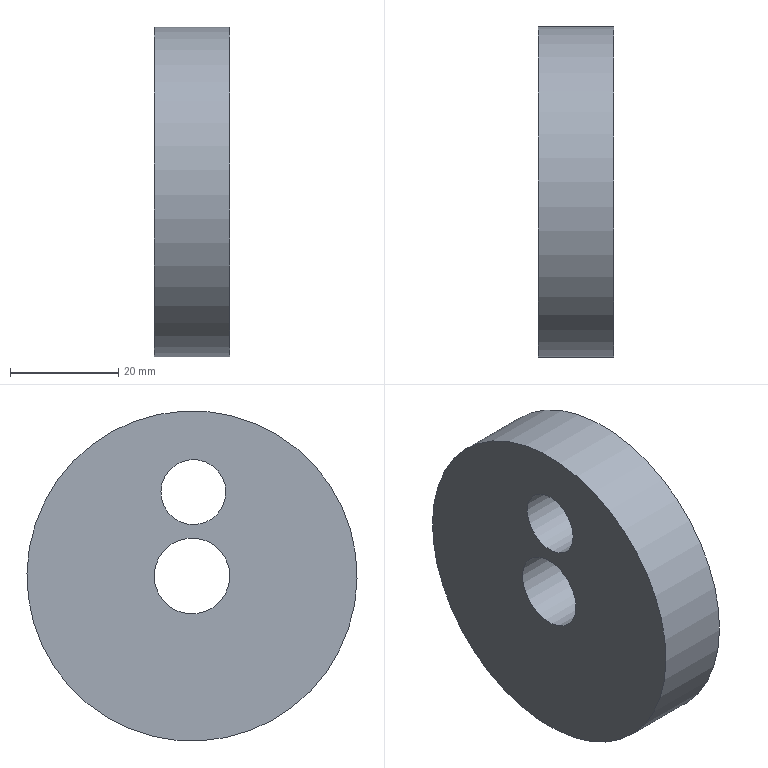Component | NX | CONNECTING_PLATE | 1 solid | 5 faces | box 14 x 61 x 61 mm | volume 37176 mm3 | cylinder 3 | plane 2 | commonest cylinder face diameters 12 x1 61 x1 14 x1
STEP:
#1=CARTESIAN_POINT('',(0.,0.,0.));
#2=DIRECTION('',(0.,0.,1.));
#3=DIRECTION('',(1.,0.,0.));
#4=AXIS2_PLACEMENT_3D('',#1,#2,#3);
#5=CARTESIAN_POINT('',(-95.,-6.249,138.401));
#6=VERTEX_POINT('',#5);
#7=CARTESIAN_POINT('',(-95.,-0.25,138.498));
#8=DIRECTION('',(-1.,0.,0.));
#9=DIRECTION('',(0.,-0.9999,-0.01613));
#10=AXIS2_PLACEMENT_3D('',#7,#8,#9);
#11=CIRCLE('',#10,6.);
#12=CARTESIAN_POINT('',(-95.,-0.25,138.498));
#13=DIRECTION('',(1.,0.,0.));
#14=DIRECTION('',(0.,0.9999,0.01613));
#15=AXIS2_PLACEMENT_3D('',#12,#13,#14);
#16=CYLINDRICAL_SURFACE('',#15,6.);
#17=CARTESIAN_POINT('',(9.425,0.));
#18=DIRECTION('',(-1.,0.));
#19=VECTOR('',#18,1.);
#20=LINE('',#17,#19);
#21=(GEOMETRIC_REPRESENTATION_CONTEXT(2)PARAMETRIC_REPRESENTATION_CONTEXT()REPRESENTATION_CONTEXT('',''));
#22=DEFINITIONAL_REPRESENTATION('',(#20),#21);
#23=PCURVE('',#16,#22);
#24=CARTESIAN_POINT('',(-95.,-0.125,130.749));
#25=DIRECTION('',(-1.,0.,0.));
#26=DIRECTION('',(0.,-0.9999,-0.01613));
#27=AXIS2_PLACEMENT_3D('',#24,#25,#26);
#28=PLANE('',#27);
#29=CARTESIAN_POINT('',(0.,7.75));
#30=DIRECTION('',(1.,-0.));
#31=AXIS2_PLACEMENT_2D('',#29,#30);
#32=CIRCLE('',#31,6.);
#33=(GEOMETRIC_REPRESENTATION_CONTEXT(2)PARAMETRIC_REPRESENTATION_CONTEXT()REPRESENTATION_CONTEXT('',''));
#34=DEFINITIONAL_REPRESENTATION('',(#32),#33);
#35=PCURVE('',#28,#34);
#36=SURFACE_CURVE('',#11,(#23,#35),.PCURVE_S1.);
#37=EDGE_CURVE('',#6,#6,#36,.T.);
#38=ORIENTED_EDGE('',*,*,#37,.F.);
#39=CARTESIAN_POINT('',(-81.,-6.249,138.401));
#40=VERTEX_POINT('',#39);
#41=CARTESIAN_POINT('',(-95.,-6.249,138.401));
#42=CARTESIAN_POINT('',(-81.,-6.249,138.401));
#43=B_SPLINE_CURVE_WITH_KNOTS('',1,(#41,#42),.UNSPECIFIED.,.F.,.F.,(2,2),(0.,14.),.PIECEWISE_BEZIER_KNOTS.);
#44=CARTESIAN_POINT('',(9.425,0.));
#45=DIRECTION('',(0.,1.));
#46=VECTOR('',#45,1.);
#47=LINE('',#44,#46);
#48=(GEOMETRIC_REPRESENTATION_CONTEXT(2)PARAMETRIC_REPRESENTATION_CONTEXT()REPRESENTATION_CONTEXT('',''));
#49=DEFINITIONAL_REPRESENTATION('',(#47),#48);
#50=PCURVE('',#16,#49);
#51=CARTESIAN_POINT('',(3.142,0.));
#52=DIRECTION('',(0.,1.));
#53=VECTOR('',#52,1.);
#54=LINE('',#51,#53);
#55=(GEOMETRIC_REPRESENTATION_CONTEXT(2)PARAMETRIC_REPRESENTATION_CONTEXT()REPRESENTATION_CONTEXT('',''));
#56=DEFINITIONAL_REPRESENTATION('',(#54),#55);
#57=PCURVE('',#16,#56);
#58=SEAM_CURVE('',#43,(#50,#57),.PCURVE_S1.);
#59=EDGE_CURVE('',#6,#40,#58,.T.);
#60=ORIENTED_EDGE('',*,*,#59,.T.);
#61=CARTESIAN_POINT('',(-81.,-0.25,138.498));
#62=DIRECTION('',(-1.,0.,0.));
#63=DIRECTION('',(0.,-0.9999,-0.01613));
#64=AXIS2_PLACEMENT_3D('',#61,#62,#63);
#65=CIRCLE('',#64,6.);
#66=CARTESIAN_POINT('',(9.425,14.));
#67=DIRECTION('',(-1.,0.));
#68=VECTOR('',#67,1.);
#69=LINE('',#66,#68);
#70=(GEOMETRIC_REPRESENTATION_CONTEXT(2)PARAMETRIC_REPRESENTATION_CONTEXT()REPRESENTATION_CONTEXT('',''));
#71=DEFINITIONAL_REPRESENTATION('',(#69),#70);
#72=PCURVE('',#16,#71);
#73=CARTESIAN_POINT('',(-81.,-0.125,130.749));
#74=DIRECTION('',(-1.,0.,0.));
#75=DIRECTION('',(0.,-0.9999,-0.01613));
#76=AXIS2_PLACEMENT_3D('',#73,#74,#75);
#77=PLANE('',#76);
#78=CARTESIAN_POINT('',(0.,7.75));
#79=DIRECTION('',(1.,-0.));
#80=AXIS2_PLACEMENT_2D('',#78,#79);
#81=CIRCLE('',#80,6.);
#82=(GEOMETRIC_REPRESENTATION_CONTEXT(2)PARAMETRIC_REPRESENTATION_CONTEXT()REPRESENTATION_CONTEXT('',''));
#83=DEFINITIONAL_REPRESENTATION('',(#81),#82);
#84=PCURVE('',#77,#83);
#85=SURFACE_CURVE('',#65,(#72,#84),.PCURVE_S1.);
#86=EDGE_CURVE('',#40,#40,#85,.T.);
#87=ORIENTED_EDGE('',*,*,#86,.T.);
#88=ORIENTED_EDGE('',*,*,#59,.F.);
#89=EDGE_LOOP('',(#38,#60,#87,#88));
#90=FACE_BOUND('',#89,.F.);
#91=ADVANCED_FACE('',(#90),#16,.F.);
#92=CARTESIAN_POINT('',(-95.,-30.496,122.508));
#93=VERTEX_POINT('',#92);
#94=CARTESIAN_POINT('',(-95.,-0.,123.));
#95=DIRECTION('',(-1.,0.,0.));
#96=DIRECTION('',(0.,-0.9999,-0.01613));
#97=AXIS2_PLACEMENT_3D('',#94,#95,#96);
#98=CIRCLE('',#97,30.5);
#99=CARTESIAN_POINT('',(-95.,-0.,123.));
#100=DIRECTION('',(1.,0.,0.));
#101=DIRECTION('',(0.,0.9999,0.01613));
#102=AXIS2_PLACEMENT_3D('',#99,#100,#101);
#103=CYLINDRICAL_SURFACE('',#102,30.5);
#104=CARTESIAN_POINT('',(9.425,0.));
#105=DIRECTION('',(-1.,0.));
#106=VECTOR('',#105,1.);
#107=LINE('',#104,#106);
#108=(GEOMETRIC_REPRESENTATION_CONTEXT(2)PARAMETRIC_REPRESENTATION_CONTEXT()REPRESENTATION_CONTEXT('',''));
#109=DEFINITIONAL_REPRESENTATION('',(#107),#108);
#110=PCURVE('',#103,#109);
#111=CARTESIAN_POINT('',(0.,-7.75));
#112=DIRECTION('',(1.,0.));
#113=AXIS2_PLACEMENT_2D('',#111,#112);
#114=CIRCLE('',#113,30.5);
#115=(GEOMETRIC_REPRESENTATION_CONTEXT(2)PARAMETRIC_REPRESENTATION_CONTEXT()REPRESENTATION_CONTEXT('',''));
#116=DEFINITIONAL_REPRESENTATION('',(#114),#115);
#117=PCURVE('',#28,#116);
#118=SURFACE_CURVE('',#98,(#110,#117),.PCURVE_S1.);
#119=EDGE_CURVE('',#93,#93,#118,.T.);
#120=ORIENTED_EDGE('',*,*,#119,.F.);
#121=CARTESIAN_POINT('',(-81.,-30.496,122.508));
#122=VERTEX_POINT('',#121);
#123=CARTESIAN_POINT('',(-95.,-30.496,122.508));
#124=CARTESIAN_POINT('',(-81.,-30.496,122.508));
#125=B_SPLINE_CURVE_WITH_KNOTS('',1,(#123,#124),.UNSPECIFIED.,.F.,.F.,(2,2),(0.,14.),.PIECEWISE_BEZIER_KNOTS.);
#126=CARTESIAN_POINT('',(9.425,0.));
#127=DIRECTION('',(0.,1.));
#128=VECTOR('',#127,1.);
#129=LINE('',#126,#128);
#130=(GEOMETRIC_REPRESENTATION_CONTEXT(2)PARAMETRIC_REPRESENTATION_CONTEXT()REPRESENTATION_CONTEXT('',''));
#131=DEFINITIONAL_REPRESENTATION('',(#129),#130);
#132=PCURVE('',#103,#131);
#133=CARTESIAN_POINT('',(3.142,0.));
#134=DIRECTION('',(0.,1.));
#135=VECTOR('',#134,1.);
#136=LINE('',#133,#135);
#137=(GEOMETRIC_REPRESENTATION_CONTEXT(2)PARAMETRIC_REPRESENTATION_CONTEXT()REPRESENTATION_CONTEXT('',''));
#138=DEFINITIONAL_REPRESENTATION('',(#136),#137);
#139=PCURVE('',#103,#138);
#140=SEAM_CURVE('',#125,(#132,#139),.PCURVE_S1.);
#141=EDGE_CURVE('',#93,#122,#140,.T.);
#142=ORIENTED_EDGE('',*,*,#141,.T.);
#143=CARTESIAN_POINT('',(-81.,-0.,123.));
#144=DIRECTION('',(-1.,0.,0.));
#145=DIRECTION('',(0.,-0.9999,-0.01613));
#146=AXIS2_PLACEMENT_3D('',#143,#144,#145);
#147=CIRCLE('',#146,30.5);
#148=CARTESIAN_POINT('',(9.425,14.));
#149=DIRECTION('',(-1.,0.));
#150=VECTOR('',#149,1.);
#151=LINE('',#148,#150);
#152=(GEOMETRIC_REPRESENTATION_CONTEXT(2)PARAMETRIC_REPRESENTATION_CONTEXT()REPRESENTATION_CONTEXT('',''));
#153=DEFINITIONAL_REPRESENTATION('',(#151),#152);
#154=PCURVE('',#103,#153);
#155=CARTESIAN_POINT('',(0.,-7.75));
#156=DIRECTION('',(1.,0.));
#157=AXIS2_PLACEMENT_2D('',#155,#156);
#158=CIRCLE('',#157,30.5);
#159=(GEOMETRIC_REPRESENTATION_CONTEXT(2)PARAMETRIC_REPRESENTATION_CONTEXT()REPRESENTATION_CONTEXT('',''));
#160=DEFINITIONAL_REPRESENTATION('',(#158),#159);
#161=PCURVE('',#77,#160);
#162=SURFACE_CURVE('',#147,(#154,#161),.PCURVE_S1.);
#163=EDGE_CURVE('',#122,#122,#162,.T.);
#164=ORIENTED_EDGE('',*,*,#163,.T.);
#165=ORIENTED_EDGE('',*,*,#141,.F.);
#166=EDGE_LOOP('',(#120,#142,#164,#165));
#167=FACE_BOUND('',#166,.T.);
#168=ADVANCED_FACE('',(#167),#103,.T.);
#169=CARTESIAN_POINT('',(-95.,-6.999,122.887));
#170=VERTEX_POINT('',#169);
#171=CARTESIAN_POINT('',(-95.,-0.,123.));
#172=DIRECTION('',(-1.,0.,0.));
#173=DIRECTION('',(0.,-0.9999,-0.01613));
#174=AXIS2_PLACEMENT_3D('',#171,#172,#173);
#175=CIRCLE('',#174,7.);
#176=CARTESIAN_POINT('',(-95.,-0.,123.));
#177=DIRECTION('',(1.,0.,0.));
#178=DIRECTION('',(0.,0.9999,0.01613));
#179=AXIS2_PLACEMENT_3D('',#176,#177,#178);
#180=CYLINDRICAL_SURFACE('',#179,7.);
#181=CARTESIAN_POINT('',(9.425,0.));
#182=DIRECTION('',(-1.,0.));
#183=VECTOR('',#182,1.);
#184=LINE('',#181,#183);
#185=(GEOMETRIC_REPRESENTATION_CONTEXT(2)PARAMETRIC_REPRESENTATION_CONTEXT()REPRESENTATION_CONTEXT('',''));
#186=DEFINITIONAL_REPRESENTATION('',(#184),#185);
#187=PCURVE('',#180,#186);
#188=CARTESIAN_POINT('',(0.,-7.75));
#189=DIRECTION('',(1.,-0.));
#190=AXIS2_PLACEMENT_2D('',#188,#189);
#191=CIRCLE('',#190,7.);
#192=(GEOMETRIC_REPRESENTATION_CONTEXT(2)PARAMETRIC_REPRESENTATION_CONTEXT()REPRESENTATION_CONTEXT('',''));
#193=DEFINITIONAL_REPRESENTATION('',(#191),#192);
#194=PCURVE('',#28,#193);
#195=SURFACE_CURVE('',#175,(#187,#194),.PCURVE_S1.);
#196=EDGE_CURVE('',#170,#170,#195,.T.);
#197=ORIENTED_EDGE('',*,*,#196,.F.);
#198=CARTESIAN_POINT('',(-81.,-6.999,122.887));
#199=VERTEX_POINT('',#198);
#200=CARTESIAN_POINT('',(-95.,-6.999,122.887));
#201=CARTESIAN_POINT('',(-81.,-6.999,122.887));
#202=B_SPLINE_CURVE_WITH_KNOTS('',1,(#200,#201),.UNSPECIFIED.,.F.,.F.,(2,2),(0.,14.),.PIECEWISE_BEZIER_KNOTS.);
#203=CARTESIAN_POINT('',(9.425,0.));
#204=DIRECTION('',(0.,1.));
#205=VECTOR('',#204,1.);
#206=LINE('',#203,#205);
#207=(GEOMETRIC_REPRESENTATION_CONTEXT(2)PARAMETRIC_REPRESENTATION_CONTEXT()REPRESENTATION_CONTEXT('',''));
#208=DEFINITIONAL_REPRESENTATION('',(#206),#207);
#209=PCURVE('',#180,#208);
#210=CARTESIAN_POINT('',(3.142,0.));
#211=DIRECTION('',(0.,1.));
#212=VECTOR('',#211,1.);
#213=LINE('',#210,#212);
#214=(GEOMETRIC_REPRESENTATION_CONTEXT(2)PARAMETRIC_REPRESENTATION_CONTEXT()REPRESENTATION_CONTEXT('',''));
#215=DEFINITIONAL_REPRESENTATION('',(#213),#214);
#216=PCURVE('',#180,#215);
#217=SEAM_CURVE('',#202,(#209,#216),.PCURVE_S1.);
#218=EDGE_CURVE('',#170,#199,#217,.T.);
#219=ORIENTED_EDGE('',*,*,#218,.T.);
#220=CARTESIAN_POINT('',(-81.,-0.,123.));
#221=DIRECTION('',(-1.,0.,0.));
#222=DIRECTION('',(0.,-0.9999,-0.01613));
#223=AXIS2_PLACEMENT_3D('',#220,#221,#222);
#224=CIRCLE('',#223,7.);
#225=CARTESIAN_POINT('',(9.425,14.));
#226=DIRECTION('',(-1.,0.));
#227=VECTOR('',#226,1.);
#228=LINE('',#225,#227);
#229=(GEOMETRIC_REPRESENTATION_CONTEXT(2)PARAMETRIC_REPRESENTATION_CONTEXT()REPRESENTATION_CONTEXT('',''));
#230=DEFINITIONAL_REPRESENTATION('',(#228),#229);
#231=PCURVE('',#180,#230);
#232=CARTESIAN_POINT('',(0.,-7.75));
#233=DIRECTION('',(1.,-0.));
#234=AXIS2_PLACEMENT_2D('',#232,#233);
#235=CIRCLE('',#234,7.);
#236=(GEOMETRIC_REPRESENTATION_CONTEXT(2)PARAMETRIC_REPRESENTATION_CONTEXT()REPRESENTATION_CONTEXT('',''));
#237=DEFINITIONAL_REPRESENTATION('',(#235),#236);
#238=PCURVE('',#77,#237);
#239=SURFACE_CURVE('',#224,(#231,#238),.PCURVE_S1.);
#240=EDGE_CURVE('',#199,#199,#239,.T.);
#241=ORIENTED_EDGE('',*,*,#240,.T.);
#242=ORIENTED_EDGE('',*,*,#218,.F.);
#243=EDGE_LOOP('',(#197,#219,#241,#242));
#244=FACE_BOUND('',#243,.F.);
#245=ADVANCED_FACE('',(#244),#180,.F.);
#246=ORIENTED_EDGE('',*,*,#119,.T.);
#247=EDGE_LOOP('',(#246));
#248=FACE_BOUND('',#247,.T.);
#249=ORIENTED_EDGE('',*,*,#37,.F.);
#250=EDGE_LOOP('',(#249));
#251=FACE_BOUND('',#250,.T.);
#252=ORIENTED_EDGE('',*,*,#196,.F.);
#253=EDGE_LOOP('',(#252));
#254=FACE_BOUND('',#253,.T.);
#255=ADVANCED_FACE('',(#248,#251,#254),#28,.T.);
#256=ORIENTED_EDGE('',*,*,#163,.F.);
#257=EDGE_LOOP('',(#256));
#258=FACE_BOUND('',#257,.T.);
#259=ORIENTED_EDGE('',*,*,#86,.T.);
#260=EDGE_LOOP('',(#259));
#261=FACE_BOUND('',#260,.T.);
#262=ORIENTED_EDGE('',*,*,#240,.T.);
#263=EDGE_LOOP('',(#262));
#264=FACE_BOUND('',#263,.T.);
#265=ADVANCED_FACE('',(#258,#261,#264),#77,.F.);
#266=CLOSED_SHELL('',(#91,#168,#245,#255,#265));
#267=MANIFOLD_SOLID_BREP('',#266);
#268=(LENGTH_UNIT()NAMED_UNIT(*)SI_UNIT(.MILLI.,.METRE.));
#269=UNCERTAINTY_MEASURE_WITH_UNIT(LENGTH_MEASURE(0.00001),#268,'','');
#270=(NAMED_UNIT(*)PLANE_ANGLE_UNIT()SI_UNIT($,.RADIAN.));
#271=(NAMED_UNIT(*)SI_UNIT($,.STERADIAN.)SOLID_ANGLE_UNIT());
#272=(GEOMETRIC_REPRESENTATION_CONTEXT(3)GLOBAL_UNCERTAINTY_ASSIGNED_CONTEXT((#269))GLOBAL_UNIT_ASSIGNED_CONTEXT((#268,#270,#271))REPRESENTATION_CONTEXT('',''));
#273=ADVANCED_BREP_SHAPE_REPRESENTATION('',(#4,#267),#272);